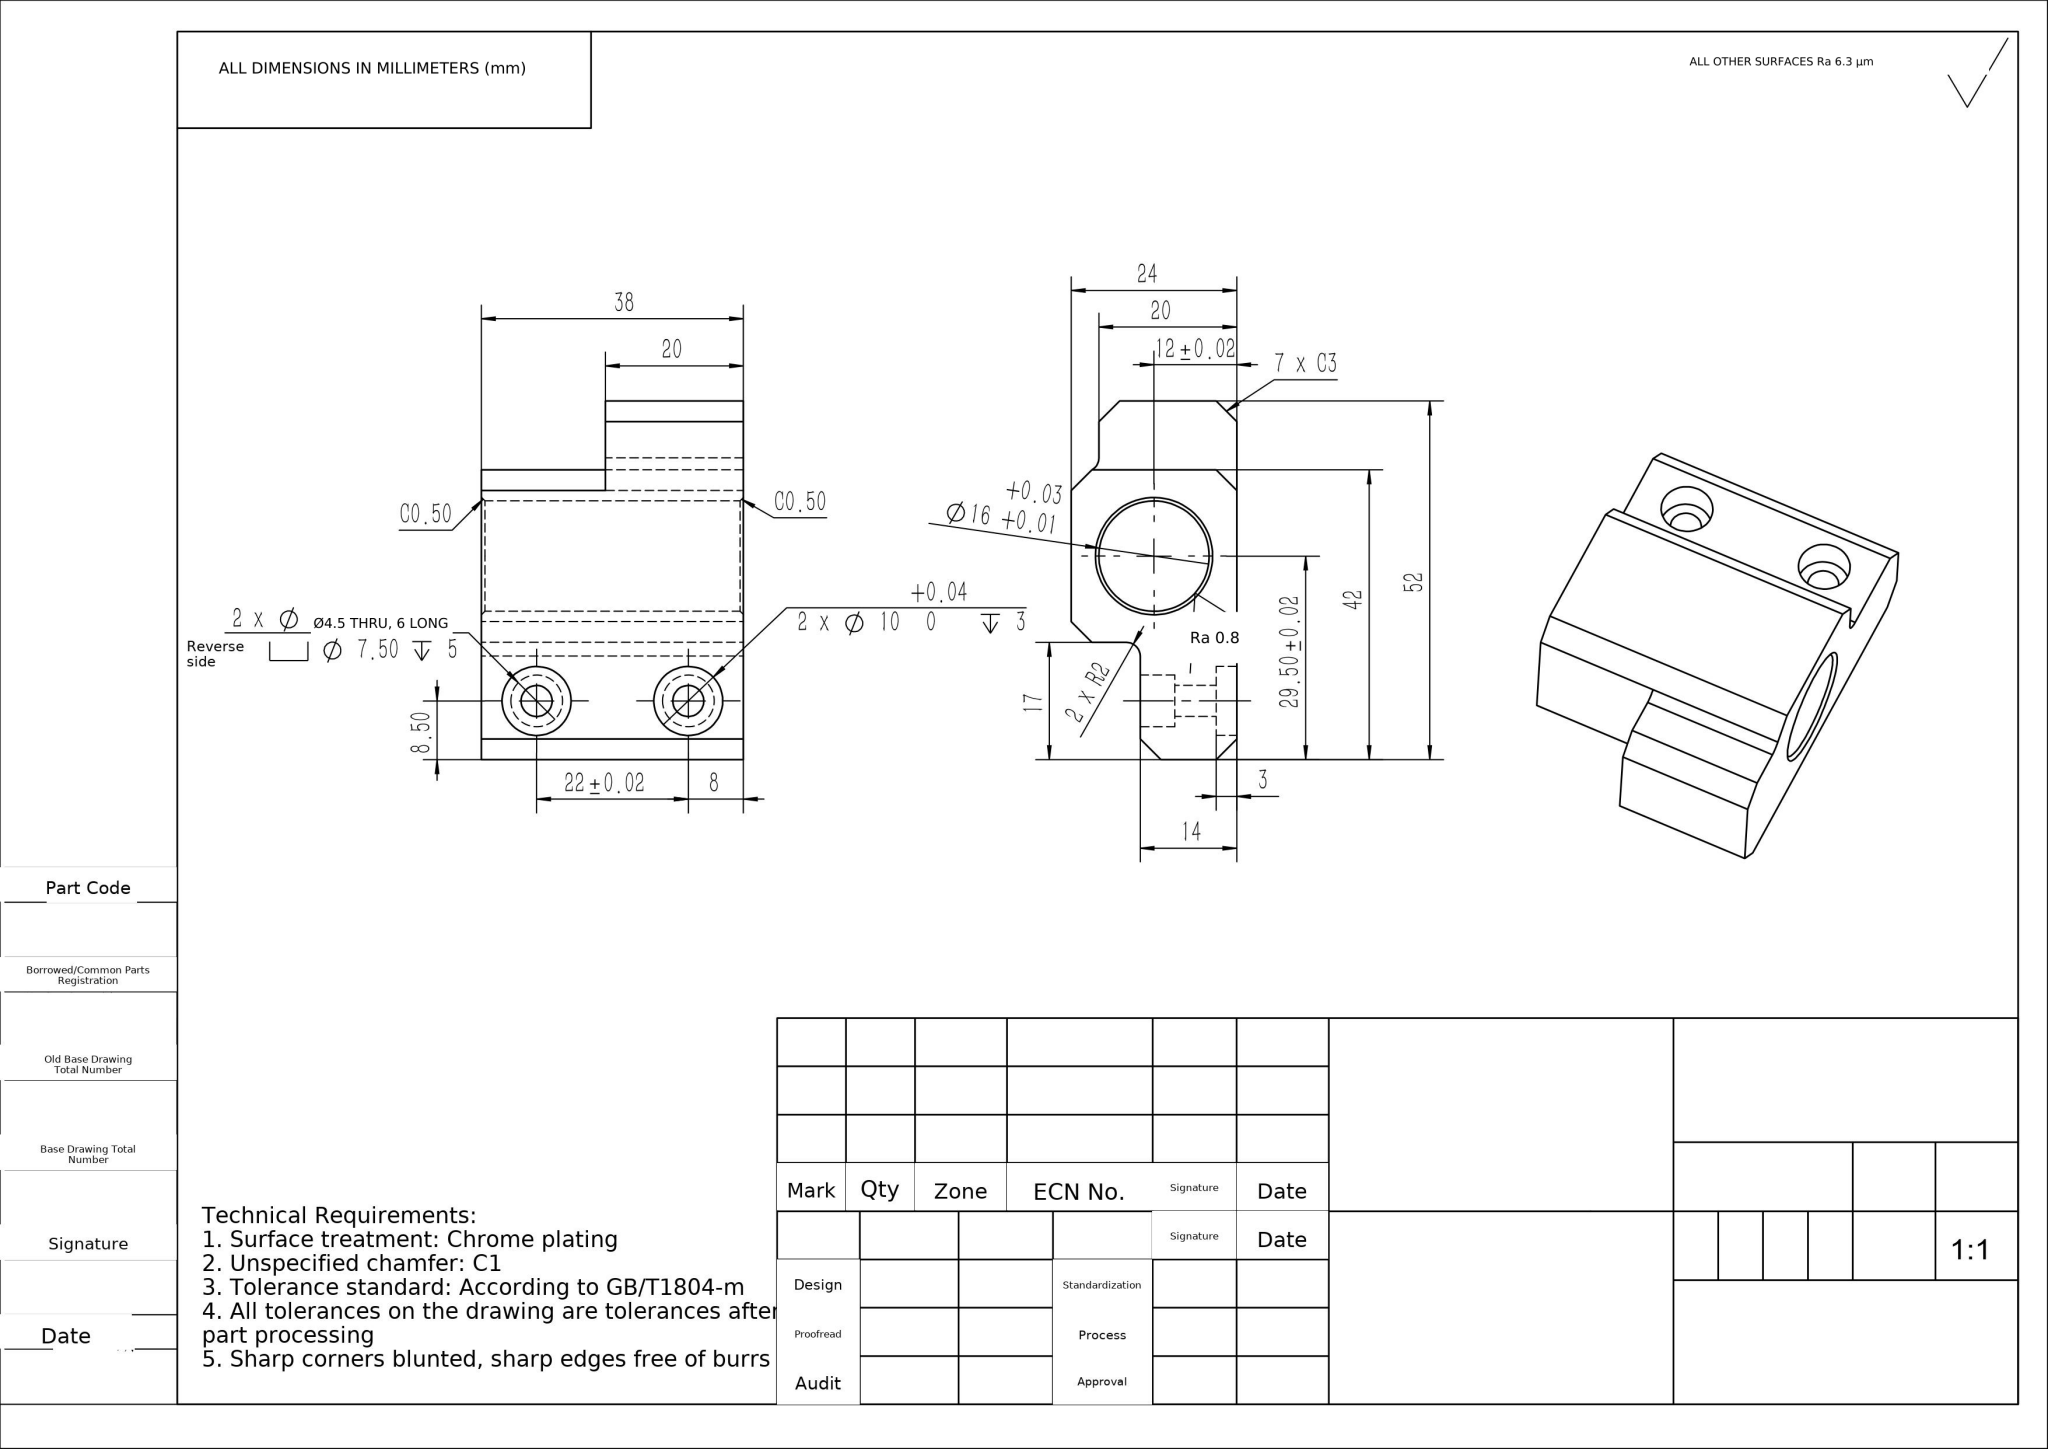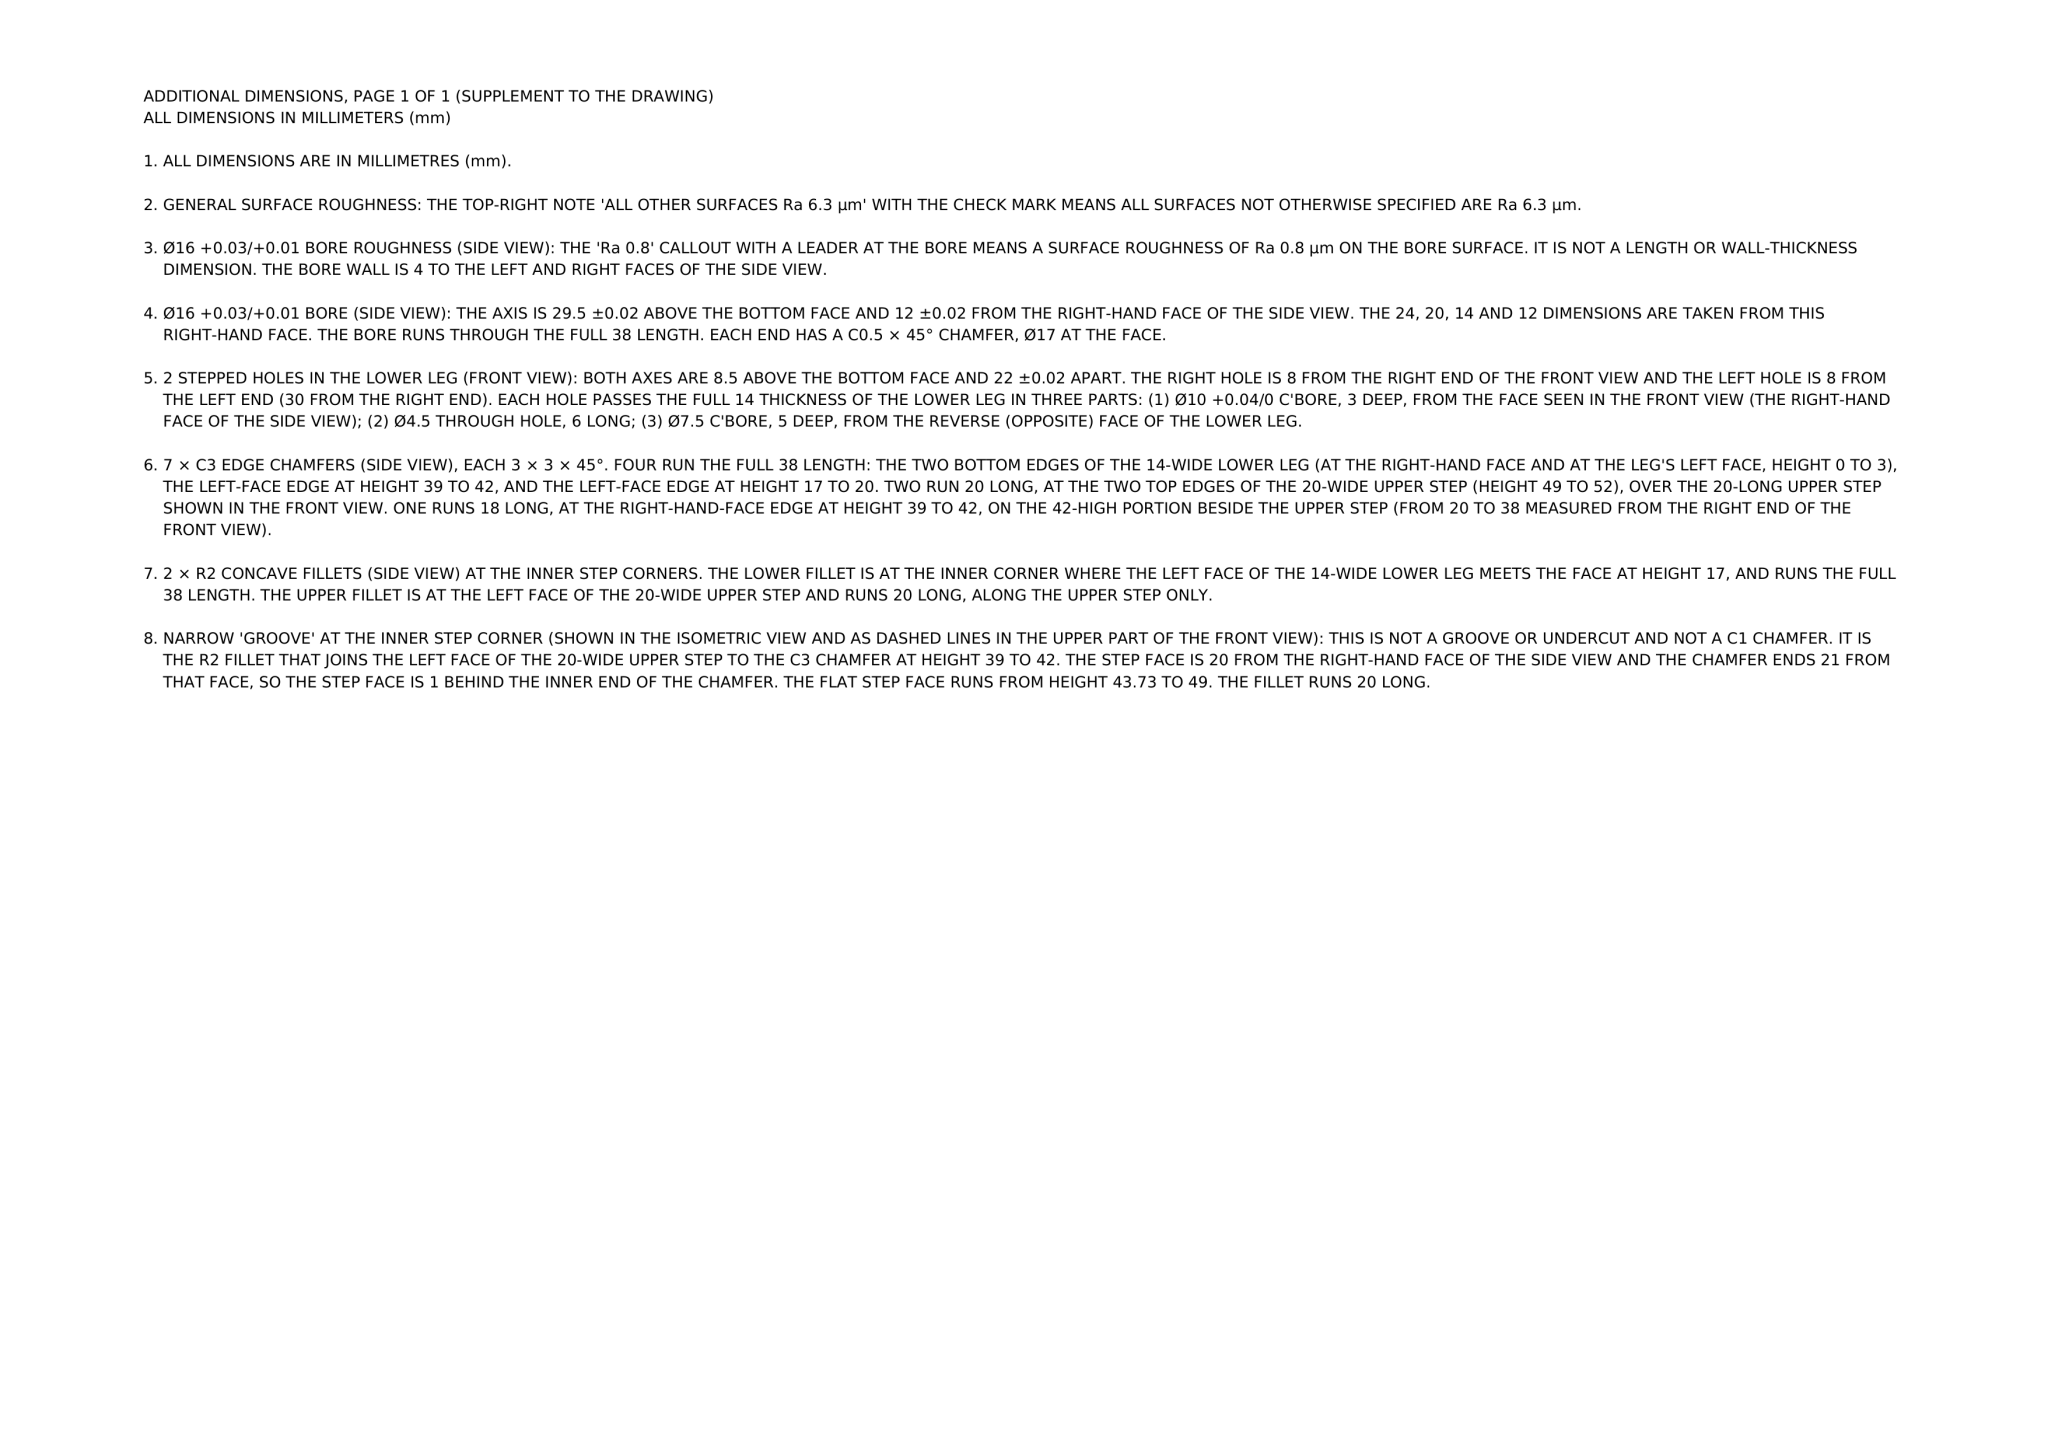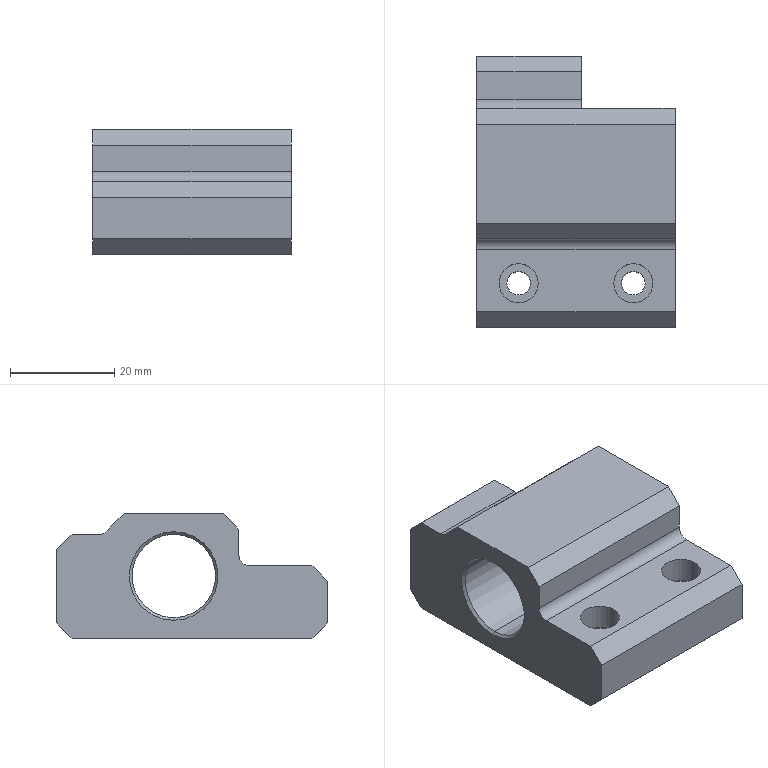Part | NX | mm | 1 solid | 42 faces | box 38 x 52 x 24 mm | volume 26185 mm3 | plane 22 | cylinder 16 | cone 4 | commonest cylinder face diameters 7.5 x4 4.5 x4 10 x4 16 x2 4 x2